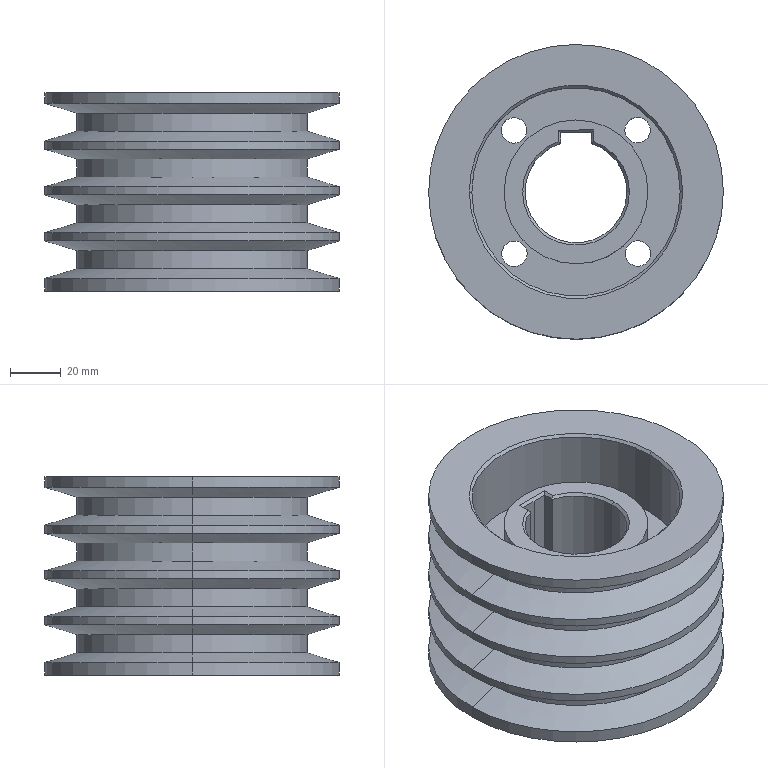Component | SolidWorks | Pulley-1 | 1 solid | 83 faces | volume 335961 mm3 | cylinder 37 | cone 26 | plane 20 | commonest cylinder face diameters 115.726 x10 90.6 x8 10 x8 56.486 x4 81.77 x4 40 x3